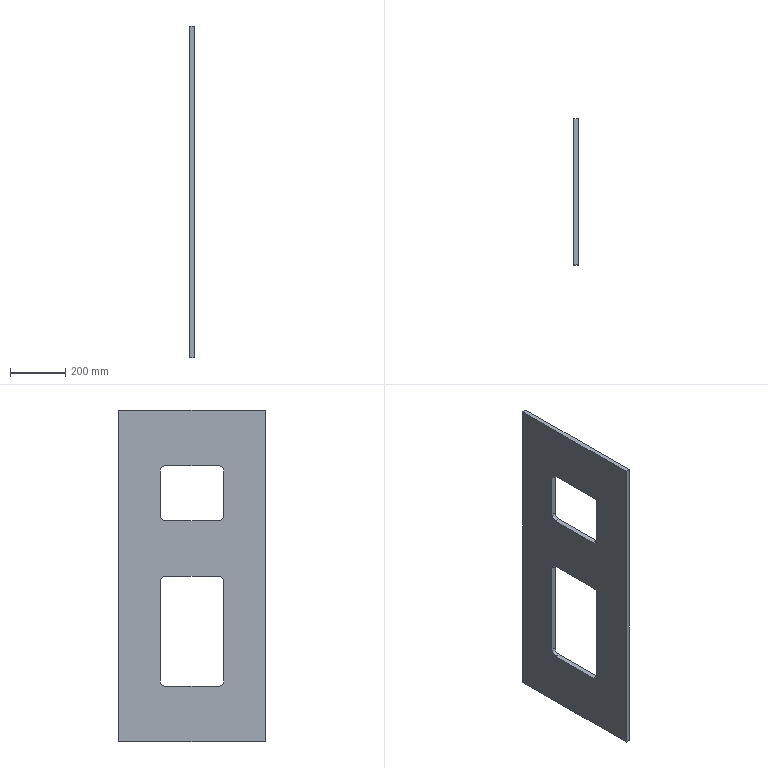Component | SolidWorks | ElectromagneticMainBeamRibPlate1-19 | 1 solid | 22 faces | box 16 x 530 x 1200 mm | volume 7978988 mm3 | plane 14 | cylinder 8 | commonest cylinder face diameters 40 x8 | material Plain Carbon Steel
STEP:
#1=COLOUR_RGB('',0.7922,0.8196,0.9333);
#2=FILL_AREA_STYLE_COLOUR('',#1);
#3=FILL_AREA_STYLE('',(#2));
#4=SURFACE_STYLE_FILL_AREA(#3);
#5=SURFACE_SIDE_STYLE('',(#4));
#6=SURFACE_STYLE_USAGE(.BOTH.,#5);
#7=PRESENTATION_STYLE_ASSIGNMENT((#6));
#8=CARTESIAN_POINT('',(-139.664,116.997,262.758));
#9=VERTEX_POINT('',#8);
#10=CARTESIAN_POINT('',(-139.664,116.997,215.514));
#11=VERTEX_POINT('',#10);
#12=CARTESIAN_POINT('',(-139.664,116.997,262.758));
#13=DIRECTION('',(-0.,0.,-1.));
#14=VECTOR('',#13,39.37);
#15=LINE('',#12,#14);
#16=EDGE_CURVE('',#9,#11,#15,.T.);
#17=ORIENTED_EDGE('',*,*,#16,.F.);
#18=CARTESIAN_POINT('',(-140.294,116.997,262.758));
#19=VERTEX_POINT('',#18);
#20=CARTESIAN_POINT('',(-140.294,116.997,262.758));
#21=DIRECTION('',(1.,0.,-0.));
#22=VECTOR('',#21,39.37);
#23=LINE('',#20,#22);
#24=EDGE_CURVE('',#19,#9,#23,.T.);
#25=ORIENTED_EDGE('',*,*,#24,.F.);
#26=CARTESIAN_POINT('',(-140.294,116.997,215.514));
#27=VERTEX_POINT('',#26);
#28=CARTESIAN_POINT('',(-140.294,116.997,262.758));
#29=DIRECTION('',(-0.,0.,-1.));
#30=VECTOR('',#29,39.37);
#31=LINE('',#28,#30);
#32=EDGE_CURVE('',#19,#27,#31,.T.);
#33=ORIENTED_EDGE('',*,*,#32,.T.);
#34=CARTESIAN_POINT('',(-140.294,116.997,215.514));
#35=DIRECTION('',(1.,0.,-0.));
#36=VECTOR('',#35,39.37);
#37=LINE('',#34,#36);
#38=EDGE_CURVE('',#27,#11,#37,.T.);
#39=ORIENTED_EDGE('',*,*,#38,.T.);
#40=EDGE_LOOP('',(#17,#25,#33,#39));
#41=FACE_OUTER_BOUND('',#40,.T.);
#42=CARTESIAN_POINT('',(-140.294,116.997,262.758));
#43=DIRECTION('',(0.,-1.,-0.));
#44=DIRECTION('',(-0.,0.,-1.));
#45=AXIS2_PLACEMENT_3D('',#42,#43,#44);
#46=PLANE('',#45);
#47=ADVANCED_FACE('',(#41),#46,.T.);
#48=CARTESIAN_POINT('',(-139.664,137.863,262.758));
#49=VERTEX_POINT('',#48);
#50=CARTESIAN_POINT('',(-139.664,116.997,262.758));
#51=DIRECTION('',(0.,-1.,0.));
#52=VECTOR('',#51,39.37);
#53=LINE('',#50,#52);
#54=EDGE_CURVE('',#49,#9,#53,.T.);
#55=ORIENTED_EDGE('',*,*,#54,.F.);
#56=CARTESIAN_POINT('',(-140.294,137.863,262.758));
#57=VERTEX_POINT('',#56);
#58=CARTESIAN_POINT('',(-140.294,137.863,262.758));
#59=DIRECTION('',(1.,0.,-0.));
#60=VECTOR('',#59,39.37);
#61=LINE('',#58,#60);
#62=EDGE_CURVE('',#57,#49,#61,.T.);
#63=ORIENTED_EDGE('',*,*,#62,.F.);
#64=CARTESIAN_POINT('',(-140.294,116.997,262.758));
#65=DIRECTION('',(0.,-1.,0.));
#66=VECTOR('',#65,39.37);
#67=LINE('',#64,#66);
#68=EDGE_CURVE('',#57,#19,#67,.T.);
#69=ORIENTED_EDGE('',*,*,#68,.T.);
#70=ORIENTED_EDGE('',*,*,#24,.T.);
#71=EDGE_LOOP('',(#55,#63,#69,#70));
#72=FACE_OUTER_BOUND('',#71,.T.);
#73=CARTESIAN_POINT('',(-140.294,116.997,262.758));
#74=DIRECTION('',(0.,0.,1.));
#75=DIRECTION('',(0.,-1.,0.));
#76=AXIS2_PLACEMENT_3D('',#73,#74,#75);
#77=PLANE('',#76);
#78=ADVANCED_FACE('',(#72),#77,.T.);
#79=CARTESIAN_POINT('',(-139.664,137.863,215.514));
#80=VERTEX_POINT('',#79);
#81=CARTESIAN_POINT('',(-139.664,137.863,262.758));
#82=DIRECTION('',(0.,-0.,1.));
#83=VECTOR('',#82,39.37);
#84=LINE('',#81,#83);
#85=EDGE_CURVE('',#80,#49,#84,.T.);
#86=ORIENTED_EDGE('',*,*,#85,.F.);
#87=CARTESIAN_POINT('',(-140.294,137.863,215.514));
#88=VERTEX_POINT('',#87);
#89=CARTESIAN_POINT('',(-140.294,137.863,215.514));
#90=DIRECTION('',(1.,0.,-0.));
#91=VECTOR('',#90,39.37);
#92=LINE('',#89,#91);
#93=EDGE_CURVE('',#88,#80,#92,.T.);
#94=ORIENTED_EDGE('',*,*,#93,.F.);
#95=CARTESIAN_POINT('',(-140.294,137.863,262.758));
#96=DIRECTION('',(0.,-0.,1.));
#97=VECTOR('',#96,39.37);
#98=LINE('',#95,#97);
#99=EDGE_CURVE('',#88,#57,#98,.T.);
#100=ORIENTED_EDGE('',*,*,#99,.T.);
#101=ORIENTED_EDGE('',*,*,#62,.T.);
#102=EDGE_LOOP('',(#86,#94,#100,#101));
#103=FACE_OUTER_BOUND('',#102,.T.);
#104=CARTESIAN_POINT('',(-140.294,137.863,262.758));
#105=DIRECTION('',(-0.,1.,0.));
#106=DIRECTION('',(0.,-0.,1.));
#107=AXIS2_PLACEMENT_3D('',#104,#105,#106);
#108=PLANE('',#107);
#109=ADVANCED_FACE('',(#103),#108,.T.);
#110=CARTESIAN_POINT('',(-139.664,116.997,215.514));
#111=DIRECTION('',(-0.,1.,0.));
#112=VECTOR('',#111,39.37);
#113=LINE('',#110,#112);
#114=EDGE_CURVE('',#11,#80,#113,.T.);
#115=ORIENTED_EDGE('',*,*,#114,.F.);
#116=ORIENTED_EDGE('',*,*,#38,.F.);
#117=CARTESIAN_POINT('',(-140.294,116.997,215.514));
#118=DIRECTION('',(-0.,1.,0.));
#119=VECTOR('',#118,39.37);
#120=LINE('',#117,#119);
#121=EDGE_CURVE('',#27,#88,#120,.T.);
#122=ORIENTED_EDGE('',*,*,#121,.T.);
#123=ORIENTED_EDGE('',*,*,#93,.T.);
#124=EDGE_LOOP('',(#115,#116,#122,#123));
#125=FACE_OUTER_BOUND('',#124,.T.);
#126=CARTESIAN_POINT('',(-140.294,116.997,215.514));
#127=DIRECTION('',(-0.,-0.,-1.));
#128=DIRECTION('',(-0.,1.,0.));
#129=AXIS2_PLACEMENT_3D('',#126,#127,#128);
#130=PLANE('',#129);
#131=ADVANCED_FACE('',(#125),#130,.T.);
#132=CARTESIAN_POINT('',(-140.294,122.903,254.096));
#133=VERTEX_POINT('',#132);
#134=CARTESIAN_POINT('',(-140.294,122.903,247.797));
#135=VERTEX_POINT('',#134);
#136=CARTESIAN_POINT('',(-140.294,122.903,254.096));
#137=DIRECTION('',(-0.,-0.,-1.));
#138=VECTOR('',#137,39.37);
#139=LINE('',#136,#138);
#140=EDGE_CURVE('',#133,#135,#139,.T.);
#141=ORIENTED_EDGE('',*,*,#140,.T.);
#142=CARTESIAN_POINT('',(-140.294,123.69,247.01));
#143=VERTEX_POINT('',#142);
#144=CARTESIAN_POINT('',(-140.294,123.69,247.797));
#145=DIRECTION('',(1.,0.,-0.));
#146=DIRECTION('',(0.,0.,-1.));
#147=AXIS2_PLACEMENT_3D('',#144,#145,#146);
#148=CIRCLE('',#147,0.7874);
#149=EDGE_CURVE('',#135,#143,#148,.T.);
#150=ORIENTED_EDGE('',*,*,#149,.T.);
#151=CARTESIAN_POINT('',(-140.294,131.171,247.01));
#152=VERTEX_POINT('',#151);
#153=CARTESIAN_POINT('',(-140.294,123.69,247.01));
#154=DIRECTION('',(-0.,1.,0.));
#155=VECTOR('',#154,39.37);
#156=LINE('',#153,#155);
#157=EDGE_CURVE('',#143,#152,#156,.T.);
#158=ORIENTED_EDGE('',*,*,#157,.T.);
#159=CARTESIAN_POINT('',(-140.294,131.958,247.797));
#160=VERTEX_POINT('',#159);
#161=CARTESIAN_POINT('',(-140.294,131.171,247.797));
#162=DIRECTION('',(1.,0.,-0.));
#163=DIRECTION('',(0.,0.,-1.));
#164=AXIS2_PLACEMENT_3D('',#161,#162,#163);
#165=CIRCLE('',#164,0.7874);
#166=EDGE_CURVE('',#152,#160,#165,.T.);
#167=ORIENTED_EDGE('',*,*,#166,.T.);
#168=CARTESIAN_POINT('',(-140.294,131.958,254.096));
#169=VERTEX_POINT('',#168);
#170=CARTESIAN_POINT('',(-140.294,131.958,254.096));
#171=DIRECTION('',(0.,0.,1.));
#172=VECTOR('',#171,39.37);
#173=LINE('',#170,#172);
#174=EDGE_CURVE('',#160,#169,#173,.T.);
#175=ORIENTED_EDGE('',*,*,#174,.T.);
#176=CARTESIAN_POINT('',(-140.294,131.171,254.884));
#177=VERTEX_POINT('',#176);
#178=CARTESIAN_POINT('',(-140.294,131.171,254.096));
#179=DIRECTION('',(1.,0.,-0.));
#180=DIRECTION('',(0.,0.,1.));
#181=AXIS2_PLACEMENT_3D('',#178,#179,#180);
#182=CIRCLE('',#181,0.7874);
#183=EDGE_CURVE('',#169,#177,#182,.T.);
#184=ORIENTED_EDGE('',*,*,#183,.T.);
#185=CARTESIAN_POINT('',(-140.294,123.69,254.884));
#186=VERTEX_POINT('',#185);
#187=CARTESIAN_POINT('',(-140.294,123.69,254.884));
#188=DIRECTION('',(0.,-1.,0.));
#189=VECTOR('',#188,39.37);
#190=LINE('',#187,#189);
#191=EDGE_CURVE('',#177,#186,#190,.T.);
#192=ORIENTED_EDGE('',*,*,#191,.T.);
#193=CARTESIAN_POINT('',(-140.294,123.69,254.096));
#194=DIRECTION('',(1.,0.,-0.));
#195=DIRECTION('',(0.,0.,-1.));
#196=AXIS2_PLACEMENT_3D('',#193,#194,#195);
#197=CIRCLE('',#196,0.7874);
#198=EDGE_CURVE('',#186,#133,#197,.T.);
#199=ORIENTED_EDGE('',*,*,#198,.T.);
#200=EDGE_LOOP('',(#141,#150,#158,#167,#175,#184,#192,#199));
#201=FACE_BOUND('',#200,.T.);
#202=CARTESIAN_POINT('',(-140.294,122.903,238.348));
#203=VERTEX_POINT('',#202);
#204=CARTESIAN_POINT('',(-140.294,122.903,224.175));
#205=VERTEX_POINT('',#204);
#206=CARTESIAN_POINT('',(-140.294,122.903,238.348));
#207=DIRECTION('',(-0.,0.,-1.));
#208=VECTOR('',#207,39.37);
#209=LINE('',#206,#208);
#210=EDGE_CURVE('',#203,#205,#209,.T.);
#211=ORIENTED_EDGE('',*,*,#210,.T.);
#212=CARTESIAN_POINT('',(-140.294,123.69,223.388));
#213=VERTEX_POINT('',#212);
#214=CARTESIAN_POINT('',(-140.294,123.69,224.175));
#215=DIRECTION('',(1.,0.,-0.));
#216=DIRECTION('',(0.,0.,-1.));
#217=AXIS2_PLACEMENT_3D('',#214,#215,#216);
#218=CIRCLE('',#217,0.7874);
#219=EDGE_CURVE('',#205,#213,#218,.T.);
#220=ORIENTED_EDGE('',*,*,#219,.T.);
#221=CARTESIAN_POINT('',(-140.294,131.171,223.388));
#222=VERTEX_POINT('',#221);
#223=CARTESIAN_POINT('',(-140.294,123.69,223.388));
#224=DIRECTION('',(-0.,1.,0.));
#225=VECTOR('',#224,39.37);
#226=LINE('',#223,#225);
#227=EDGE_CURVE('',#213,#222,#226,.T.);
#228=ORIENTED_EDGE('',*,*,#227,.T.);
#229=CARTESIAN_POINT('',(-140.294,131.958,224.175));
#230=VERTEX_POINT('',#229);
#231=CARTESIAN_POINT('',(-140.294,131.171,224.175));
#232=DIRECTION('',(1.,0.,-0.));
#233=DIRECTION('',(0.,0.,-1.));
#234=AXIS2_PLACEMENT_3D('',#231,#232,#233);
#235=CIRCLE('',#234,0.7874);
#236=EDGE_CURVE('',#222,#230,#235,.T.);
#237=ORIENTED_EDGE('',*,*,#236,.T.);
#238=CARTESIAN_POINT('',(-140.294,131.958,238.348));
#239=VERTEX_POINT('',#238);
#240=CARTESIAN_POINT('',(-140.294,131.958,238.348));
#241=DIRECTION('',(0.,0.,1.));
#242=VECTOR('',#241,39.37);
#243=LINE('',#240,#242);
#244=EDGE_CURVE('',#230,#239,#243,.T.);
#245=ORIENTED_EDGE('',*,*,#244,.T.);
#246=CARTESIAN_POINT('',(-140.294,131.171,239.136));
#247=VERTEX_POINT('',#246);
#248=CARTESIAN_POINT('',(-140.294,131.171,238.348));
#249=DIRECTION('',(1.,0.,-0.));
#250=DIRECTION('',(0.,0.,1.));
#251=AXIS2_PLACEMENT_3D('',#248,#249,#250);
#252=CIRCLE('',#251,0.7874);
#253=EDGE_CURVE('',#239,#247,#252,.T.);
#254=ORIENTED_EDGE('',*,*,#253,.T.);
#255=CARTESIAN_POINT('',(-140.294,123.69,239.136));
#256=VERTEX_POINT('',#255);
#257=CARTESIAN_POINT('',(-140.294,123.69,239.136));
#258=DIRECTION('',(0.,-1.,0.));
#259=VECTOR('',#258,39.37);
#260=LINE('',#257,#259);
#261=EDGE_CURVE('',#247,#256,#260,.T.);
#262=ORIENTED_EDGE('',*,*,#261,.T.);
#263=CARTESIAN_POINT('',(-140.294,123.69,238.348));
#264=DIRECTION('',(1.,0.,-0.));
#265=DIRECTION('',(0.,0.,-1.));
#266=AXIS2_PLACEMENT_3D('',#263,#264,#265);
#267=CIRCLE('',#266,0.7874);
#268=EDGE_CURVE('',#256,#203,#267,.T.);
#269=ORIENTED_EDGE('',*,*,#268,.T.);
#270=EDGE_LOOP('',(#211,#220,#228,#237,#245,#254,#262,#269));
#271=FACE_BOUND('',#270,.T.);
#272=ORIENTED_EDGE('',*,*,#32,.F.);
#273=ORIENTED_EDGE('',*,*,#68,.F.);
#274=ORIENTED_EDGE('',*,*,#99,.F.);
#275=ORIENTED_EDGE('',*,*,#121,.F.);
#276=EDGE_LOOP('',(#272,#273,#274,#275));
#277=FACE_OUTER_BOUND('',#276,.T.);
#278=CARTESIAN_POINT('',(-140.294,116.997,262.758));
#279=DIRECTION('',(1.,0.,-0.));
#280=DIRECTION('',(-0.,-0.,-1.));
#281=AXIS2_PLACEMENT_3D('',#278,#279,#280);
#282=PLANE('',#281);
#283=ADVANCED_FACE('',(#201,#271,#277),#282,.F.);
#284=CARTESIAN_POINT('',(-139.664,122.903,247.797));
#285=VERTEX_POINT('',#284);
#286=CARTESIAN_POINT('',(-139.664,123.69,247.01));
#287=VERTEX_POINT('',#286);
#288=CARTESIAN_POINT('',(-139.664,123.69,247.797));
#289=DIRECTION('',(1.,0.,-0.));
#290=DIRECTION('',(0.,0.,-1.));
#291=AXIS2_PLACEMENT_3D('',#288,#289,#290);
#292=CIRCLE('',#291,0.7874);
#293=EDGE_CURVE('',#285,#287,#292,.T.);
#294=ORIENTED_EDGE('',*,*,#293,.F.);
#295=CARTESIAN_POINT('',(-139.664,122.903,254.096));
#296=VERTEX_POINT('',#295);
#297=CARTESIAN_POINT('',(-139.664,122.903,254.096));
#298=DIRECTION('',(-0.,-0.,-1.));
#299=VECTOR('',#298,39.37);
#300=LINE('',#297,#299);
#301=EDGE_CURVE('',#296,#285,#300,.T.);
#302=ORIENTED_EDGE('',*,*,#301,.F.);
#303=CARTESIAN_POINT('',(-139.664,123.69,254.884));
#304=VERTEX_POINT('',#303);
#305=CARTESIAN_POINT('',(-139.664,123.69,254.096));
#306=DIRECTION('',(1.,0.,-0.));
#307=DIRECTION('',(0.,0.,-1.));
#308=AXIS2_PLACEMENT_3D('',#305,#306,#307);
#309=CIRCLE('',#308,0.7874);
#310=EDGE_CURVE('',#304,#296,#309,.T.);
#311=ORIENTED_EDGE('',*,*,#310,.F.);
#312=CARTESIAN_POINT('',(-139.664,131.171,254.884));
#313=VERTEX_POINT('',#312);
#314=CARTESIAN_POINT('',(-139.664,123.69,254.884));
#315=DIRECTION('',(0.,-1.,0.));
#316=VECTOR('',#315,39.37);
#317=LINE('',#314,#316);
#318=EDGE_CURVE('',#313,#304,#317,.T.);
#319=ORIENTED_EDGE('',*,*,#318,.F.);
#320=CARTESIAN_POINT('',(-139.664,131.958,254.096));
#321=VERTEX_POINT('',#320);
#322=CARTESIAN_POINT('',(-139.664,131.171,254.096));
#323=DIRECTION('',(1.,0.,-0.));
#324=DIRECTION('',(0.,0.,1.));
#325=AXIS2_PLACEMENT_3D('',#322,#323,#324);
#326=CIRCLE('',#325,0.7874);
#327=EDGE_CURVE('',#321,#313,#326,.T.);
#328=ORIENTED_EDGE('',*,*,#327,.F.);
#329=CARTESIAN_POINT('',(-139.664,131.958,247.797));
#330=VERTEX_POINT('',#329);
#331=CARTESIAN_POINT('',(-139.664,131.958,254.096));
#332=DIRECTION('',(0.,0.,1.));
#333=VECTOR('',#332,39.37);
#334=LINE('',#331,#333);
#335=EDGE_CURVE('',#330,#321,#334,.T.);
#336=ORIENTED_EDGE('',*,*,#335,.F.);
#337=CARTESIAN_POINT('',(-139.664,131.171,247.01));
#338=VERTEX_POINT('',#337);
#339=CARTESIAN_POINT('',(-139.664,131.171,247.797));
#340=DIRECTION('',(1.,0.,-0.));
#341=DIRECTION('',(0.,0.,-1.));
#342=AXIS2_PLACEMENT_3D('',#339,#340,#341);
#343=CIRCLE('',#342,0.7874);
#344=EDGE_CURVE('',#338,#330,#343,.T.);
#345=ORIENTED_EDGE('',*,*,#344,.F.);
#346=CARTESIAN_POINT('',(-139.664,123.69,247.01));
#347=DIRECTION('',(-0.,1.,0.));
#348=VECTOR('',#347,39.37);
#349=LINE('',#346,#348);
#350=EDGE_CURVE('',#287,#338,#349,.T.);
#351=ORIENTED_EDGE('',*,*,#350,.F.);
#352=EDGE_LOOP('',(#294,#302,#311,#319,#328,#336,#345,#351));
#353=FACE_BOUND('',#352,.T.);
#354=CARTESIAN_POINT('',(-139.664,122.903,224.175));
#355=VERTEX_POINT('',#354);
#356=CARTESIAN_POINT('',(-139.664,123.69,223.388));
#357=VERTEX_POINT('',#356);
#358=CARTESIAN_POINT('',(-139.664,123.69,224.175));
#359=DIRECTION('',(1.,0.,-0.));
#360=DIRECTION('',(0.,0.,-1.));
#361=AXIS2_PLACEMENT_3D('',#358,#359,#360);
#362=CIRCLE('',#361,0.7874);
#363=EDGE_CURVE('',#355,#357,#362,.T.);
#364=ORIENTED_EDGE('',*,*,#363,.F.);
#365=CARTESIAN_POINT('',(-139.664,122.903,238.348));
#366=VERTEX_POINT('',#365);
#367=CARTESIAN_POINT('',(-139.664,122.903,238.348));
#368=DIRECTION('',(-0.,0.,-1.));
#369=VECTOR('',#368,39.37);
#370=LINE('',#367,#369);
#371=EDGE_CURVE('',#366,#355,#370,.T.);
#372=ORIENTED_EDGE('',*,*,#371,.F.);
#373=CARTESIAN_POINT('',(-139.664,123.69,239.136));
#374=VERTEX_POINT('',#373);
#375=CARTESIAN_POINT('',(-139.664,123.69,238.348));
#376=DIRECTION('',(1.,0.,-0.));
#377=DIRECTION('',(0.,0.,-1.));
#378=AXIS2_PLACEMENT_3D('',#375,#376,#377);
#379=CIRCLE('',#378,0.7874);
#380=EDGE_CURVE('',#374,#366,#379,.T.);
#381=ORIENTED_EDGE('',*,*,#380,.F.);
#382=CARTESIAN_POINT('',(-139.664,131.171,239.136));
#383=VERTEX_POINT('',#382);
#384=CARTESIAN_POINT('',(-139.664,123.69,239.136));
#385=DIRECTION('',(0.,-1.,0.));
#386=VECTOR('',#385,39.37);
#387=LINE('',#384,#386);
#388=EDGE_CURVE('',#383,#374,#387,.T.);
#389=ORIENTED_EDGE('',*,*,#388,.F.);
#390=CARTESIAN_POINT('',(-139.664,131.958,238.348));
#391=VERTEX_POINT('',#390);
#392=CARTESIAN_POINT('',(-139.664,131.171,238.348));
#393=DIRECTION('',(1.,0.,-0.));
#394=DIRECTION('',(0.,0.,1.));
#395=AXIS2_PLACEMENT_3D('',#392,#393,#394);
#396=CIRCLE('',#395,0.7874);
#397=EDGE_CURVE('',#391,#383,#396,.T.);
#398=ORIENTED_EDGE('',*,*,#397,.F.);
#399=CARTESIAN_POINT('',(-139.664,131.958,224.175));
#400=VERTEX_POINT('',#399);
#401=CARTESIAN_POINT('',(-139.664,131.958,238.348));
#402=DIRECTION('',(0.,0.,1.));
#403=VECTOR('',#402,39.37);
#404=LINE('',#401,#403);
#405=EDGE_CURVE('',#400,#391,#404,.T.);
#406=ORIENTED_EDGE('',*,*,#405,.F.);
#407=CARTESIAN_POINT('',(-139.664,131.171,223.388));
#408=VERTEX_POINT('',#407);
#409=CARTESIAN_POINT('',(-139.664,131.171,224.175));
#410=DIRECTION('',(1.,0.,-0.));
#411=DIRECTION('',(0.,0.,-1.));
#412=AXIS2_PLACEMENT_3D('',#409,#410,#411);
#413=CIRCLE('',#412,0.7874);
#414=EDGE_CURVE('',#408,#400,#413,.T.);
#415=ORIENTED_EDGE('',*,*,#414,.F.);
#416=CARTESIAN_POINT('',(-139.664,123.69,223.388));
#417=DIRECTION('',(-0.,1.,0.));
#418=VECTOR('',#417,39.37);
#419=LINE('',#416,#418);
#420=EDGE_CURVE('',#357,#408,#419,.T.);
#421=ORIENTED_EDGE('',*,*,#420,.F.);
#422=EDGE_LOOP('',(#364,#372,#381,#389,#398,#406,#415,#421));
#423=FACE_BOUND('',#422,.T.);
#424=ORIENTED_EDGE('',*,*,#16,.T.);
#425=ORIENTED_EDGE('',*,*,#114,.T.);
#426=ORIENTED_EDGE('',*,*,#85,.T.);
#427=ORIENTED_EDGE('',*,*,#54,.T.);
#428=EDGE_LOOP('',(#424,#425,#426,#427));
#429=FACE_OUTER_BOUND('',#428,.T.);
#430=CARTESIAN_POINT('',(-139.664,116.997,262.758));
#431=DIRECTION('',(1.,0.,-0.));
#432=DIRECTION('',(-0.,-0.,-1.));
#433=AXIS2_PLACEMENT_3D('',#430,#431,#432);
#434=PLANE('',#433);
#435=ADVANCED_FACE('',(#353,#423,#429),#434,.T.);
#436=ORIENTED_EDGE('',*,*,#363,.T.);
#437=CARTESIAN_POINT('',(-140.294,123.69,223.388));
#438=DIRECTION('',(1.,0.,-0.));
#439=VECTOR('',#438,39.37);
#440=LINE('',#437,#439);
#441=EDGE_CURVE('',#213,#357,#440,.T.);
#442=ORIENTED_EDGE('',*,*,#441,.F.);
#443=ORIENTED_EDGE('',*,*,#219,.F.);
#444=CARTESIAN_POINT('',(-140.294,122.903,224.175));
#445=DIRECTION('',(1.,0.,-0.));
#446=VECTOR('',#445,39.37);
#447=LINE('',#444,#446);
#448=EDGE_CURVE('',#205,#355,#447,.T.);
#449=ORIENTED_EDGE('',*,*,#448,.T.);
#450=EDGE_LOOP('',(#436,#442,#443,#449));
#451=FACE_OUTER_BOUND('',#450,.T.);
#452=CARTESIAN_POINT('',(-140.294,123.69,224.175));
#453=DIRECTION('',(1.,0.,-0.));
#454=DIRECTION('',(0.,0.,-1.));
#455=AXIS2_PLACEMENT_3D('',#452,#453,#454);
#456=CYLINDRICAL_SURFACE('',#455,0.7874);
#457=ADVANCED_FACE('',(#451),#456,.F.);
#458=ORIENTED_EDGE('',*,*,#371,.T.);
#459=ORIENTED_EDGE('',*,*,#448,.F.);
#460=ORIENTED_EDGE('',*,*,#210,.F.);
#461=CARTESIAN_POINT('',(-140.294,122.903,238.348));
#462=DIRECTION('',(1.,0.,-0.));
#463=VECTOR('',#462,39.37);
#464=LINE('',#461,#463);
#465=EDGE_CURVE('',#203,#366,#464,.T.);
#466=ORIENTED_EDGE('',*,*,#465,.T.);
#467=EDGE_LOOP('',(#458,#459,#460,#466));
#468=FACE_OUTER_BOUND('',#467,.T.);
#469=CARTESIAN_POINT('',(-140.294,122.903,238.348));
#470=DIRECTION('',(0.,-1.,-0.));
#471=DIRECTION('',(-0.,0.,-1.));
#472=AXIS2_PLACEMENT_3D('',#469,#470,#471);
#473=PLANE('',#472);
#474=ADVANCED_FACE('',(#468),#473,.F.);
#475=ORIENTED_EDGE('',*,*,#380,.T.);
#476=ORIENTED_EDGE('',*,*,#465,.F.);
#477=ORIENTED_EDGE('',*,*,#268,.F.);
#478=CARTESIAN_POINT('',(-140.294,123.69,239.136));
#479=DIRECTION('',(1.,0.,-0.));
#480=VECTOR('',#479,39.37);
#481=LINE('',#478,#480);
#482=EDGE_CURVE('',#256,#374,#481,.T.);
#483=ORIENTED_EDGE('',*,*,#482,.T.);
#484=EDGE_LOOP('',(#475,#476,#477,#483));
#485=FACE_OUTER_BOUND('',#484,.T.);
#486=CARTESIAN_POINT('',(-140.294,123.69,238.348));
#487=DIRECTION('',(1.,0.,-0.));
#488=DIRECTION('',(0.,0.,-1.));
#489=AXIS2_PLACEMENT_3D('',#486,#487,#488);
#490=CYLINDRICAL_SURFACE('',#489,0.7874);
#491=ADVANCED_FACE('',(#485),#490,.F.);
#492=ORIENTED_EDGE('',*,*,#388,.T.);
#493=ORIENTED_EDGE('',*,*,#482,.F.);
#494=ORIENTED_EDGE('',*,*,#261,.F.);
#495=CARTESIAN_POINT('',(-140.294,131.171,239.136));
#496=DIRECTION('',(1.,0.,-0.));
#497=VECTOR('',#496,39.37);
#498=LINE('',#495,#497);
#499=EDGE_CURVE('',#247,#383,#498,.T.);
#500=ORIENTED_EDGE('',*,*,#499,.T.);
#501=EDGE_LOOP('',(#492,#493,#494,#500));
#502=FACE_OUTER_BOUND('',#501,.T.);
#503=CARTESIAN_POINT('',(-140.294,123.69,239.136));
#504=DIRECTION('',(0.,0.,1.));
#505=DIRECTION('',(0.,-1.,0.));
#506=AXIS2_PLACEMENT_3D('',#503,#504,#505);
#507=PLANE('',#506);
#508=ADVANCED_FACE('',(#502),#507,.F.);
#509=ORIENTED_EDGE('',*,*,#397,.T.);
#510=ORIENTED_EDGE('',*,*,#499,.F.);
#511=ORIENTED_EDGE('',*,*,#253,.F.);
#512=CARTESIAN_POINT('',(-140.294,131.958,238.348));
#513=DIRECTION('',(1.,0.,-0.));
#514=VECTOR('',#513,39.37);
#515=LINE('',#512,#514);
#516=EDGE_CURVE('',#239,#391,#515,.T.);
#517=ORIENTED_EDGE('',*,*,#516,.T.);
#518=EDGE_LOOP('',(#509,#510,#511,#517));
#519=FACE_OUTER_BOUND('',#518,.T.);
#520=CARTESIAN_POINT('',(-140.294,131.171,238.348));
#521=DIRECTION('',(1.,0.,-0.));
#522=DIRECTION('',(0.,0.,-1.));
#523=AXIS2_PLACEMENT_3D('',#520,#521,#522);
#524=CYLINDRICAL_SURFACE('',#523,0.7874);
#525=ADVANCED_FACE('',(#519),#524,.F.);
#526=ORIENTED_EDGE('',*,*,#405,.T.);
#527=ORIENTED_EDGE('',*,*,#516,.F.);
#528=ORIENTED_EDGE('',*,*,#244,.F.);
#529=CARTESIAN_POINT('',(-140.294,131.958,224.175));
#530=DIRECTION('',(1.,0.,-0.));
#531=VECTOR('',#530,39.37);
#532=LINE('',#529,#531);
#533=EDGE_CURVE('',#230,#400,#532,.T.);
#534=ORIENTED_EDGE('',*,*,#533,.T.);
#535=EDGE_LOOP('',(#526,#527,#528,#534));
#536=FACE_OUTER_BOUND('',#535,.T.);
#537=CARTESIAN_POINT('',(-140.294,131.958,238.348));
#538=DIRECTION('',(-0.,1.,-0.));
#539=DIRECTION('',(0.,0.,1.));
#540=AXIS2_PLACEMENT_3D('',#537,#538,#539);
#541=PLANE('',#540);
#542=ADVANCED_FACE('',(#536),#541,.F.);
#543=ORIENTED_EDGE('',*,*,#414,.T.);
#544=ORIENTED_EDGE('',*,*,#533,.F.);
#545=ORIENTED_EDGE('',*,*,#236,.F.);
#546=CARTESIAN_POINT('',(-140.294,131.171,223.388));
#547=DIRECTION('',(1.,0.,-0.));
#548=VECTOR('',#547,39.37);
#549=LINE('',#546,#548);
#550=EDGE_CURVE('',#222,#408,#549,.T.);
#551=ORIENTED_EDGE('',*,*,#550,.T.);
#552=EDGE_LOOP('',(#543,#544,#545,#551));
#553=FACE_OUTER_BOUND('',#552,.T.);
#554=CARTESIAN_POINT('',(-140.294,131.171,224.175));
#555=DIRECTION('',(1.,0.,-0.));
#556=DIRECTION('',(0.,0.,-1.));
#557=AXIS2_PLACEMENT_3D('',#554,#555,#556);
#558=CYLINDRICAL_SURFACE('',#557,0.7874);
#559=ADVANCED_FACE('',(#553),#558,.F.);
#560=ORIENTED_EDGE('',*,*,#420,.T.);
#561=ORIENTED_EDGE('',*,*,#550,.F.);
#562=ORIENTED_EDGE('',*,*,#227,.F.);
#563=ORIENTED_EDGE('',*,*,#441,.T.);
#564=EDGE_LOOP('',(#560,#561,#562,#563));
#565=FACE_OUTER_BOUND('',#564,.T.);
#566=CARTESIAN_POINT('',(-140.294,123.69,223.388));
#567=DIRECTION('',(-0.,-0.,-1.));
#568=DIRECTION('',(-0.,1.,0.));
#569=AXIS2_PLACEMENT_3D('',#566,#567,#568);
#570=PLANE('',#569);
#571=ADVANCED_FACE('',(#565),#570,.F.);
#572=ORIENTED_EDGE('',*,*,#293,.T.);
#573=CARTESIAN_POINT('',(-140.294,123.69,247.01));
#574=DIRECTION('',(1.,0.,-0.));
#575=VECTOR('',#574,39.37);
#576=LINE('',#573,#575);
#577=EDGE_CURVE('',#143,#287,#576,.T.);
#578=ORIENTED_EDGE('',*,*,#577,.F.);
#579=ORIENTED_EDGE('',*,*,#149,.F.);
#580=CARTESIAN_POINT('',(-140.294,122.903,247.797));
#581=DIRECTION('',(1.,0.,-0.));
#582=VECTOR('',#581,39.37);
#583=LINE('',#580,#582);
#584=EDGE_CURVE('',#135,#285,#583,.T.);
#585=ORIENTED_EDGE('',*,*,#584,.T.);
#586=EDGE_LOOP('',(#572,#578,#579,#585));
#587=FACE_OUTER_BOUND('',#586,.T.);
#588=CARTESIAN_POINT('',(-140.294,123.69,247.797));
#589=DIRECTION('',(1.,0.,-0.));
#590=DIRECTION('',(0.,0.,-1.));
#591=AXIS2_PLACEMENT_3D('',#588,#589,#590);
#592=CYLINDRICAL_SURFACE('',#591,0.7874);
#593=ADVANCED_FACE('',(#587),#592,.F.);
#594=ORIENTED_EDGE('',*,*,#301,.T.);
#595=ORIENTED_EDGE('',*,*,#584,.F.);
#596=ORIENTED_EDGE('',*,*,#140,.F.);
#597=CARTESIAN_POINT('',(-140.294,122.903,254.096));
#598=DIRECTION('',(1.,0.,-0.));
#599=VECTOR('',#598,39.37);
#600=LINE('',#597,#599);
#601=EDGE_CURVE('',#133,#296,#600,.T.);
#602=ORIENTED_EDGE('',*,*,#601,.T.);
#603=EDGE_LOOP('',(#594,#595,#596,#602));
#604=FACE_OUTER_BOUND('',#603,.T.);
#605=CARTESIAN_POINT('',(-140.294,122.903,254.096));
#606=DIRECTION('',(0.,-1.,0.));
#607=DIRECTION('',(-0.,-0.,-1.));
#608=AXIS2_PLACEMENT_3D('',#605,#606,#607);
#609=PLANE('',#608);
#610=ADVANCED_FACE('',(#604),#609,.F.);
#611=ORIENTED_EDGE('',*,*,#310,.T.);
#612=ORIENTED_EDGE('',*,*,#601,.F.);
#613=ORIENTED_EDGE('',*,*,#198,.F.);
#614=CARTESIAN_POINT('',(-140.294,123.69,254.884));
#615=DIRECTION('',(1.,0.,-0.));
#616=VECTOR('',#615,39.37);
#617=LINE('',#614,#616);
#618=EDGE_CURVE('',#186,#304,#617,.T.);
#619=ORIENTED_EDGE('',*,*,#618,.T.);
#620=EDGE_LOOP('',(#611,#612,#613,#619));
#621=FACE_OUTER_BOUND('',#620,.T.);
#622=CARTESIAN_POINT('',(-140.294,123.69,254.096));
#623=DIRECTION('',(1.,0.,-0.));
#624=DIRECTION('',(0.,0.,-1.));
#625=AXIS2_PLACEMENT_3D('',#622,#623,#624);
#626=CYLINDRICAL_SURFACE('',#625,0.7874);
#627=ADVANCED_FACE('',(#621),#626,.F.);
#628=ORIENTED_EDGE('',*,*,#318,.T.);
#629=ORIENTED_EDGE('',*,*,#618,.F.);
#630=ORIENTED_EDGE('',*,*,#191,.F.);
#631=CARTESIAN_POINT('',(-140.294,131.171,254.884));
#632=DIRECTION('',(1.,0.,-0.));
#633=VECTOR('',#632,39.37);
#634=LINE('',#631,#633);
#635=EDGE_CURVE('',#177,#313,#634,.T.);
#636=ORIENTED_EDGE('',*,*,#635,.T.);
#637=EDGE_LOOP('',(#628,#629,#630,#636));
#638=FACE_OUTER_BOUND('',#637,.T.);
#639=CARTESIAN_POINT('',(-140.294,123.69,254.884));
#640=DIRECTION('',(0.,0.,1.));
#641=DIRECTION('',(0.,-1.,0.));
#642=AXIS2_PLACEMENT_3D('',#639,#640,#641);
#643=PLANE('',#642);
#644=ADVANCED_FACE('',(#638),#643,.F.);
#645=ORIENTED_EDGE('',*,*,#327,.T.);
#646=ORIENTED_EDGE('',*,*,#635,.F.);
#647=ORIENTED_EDGE('',*,*,#183,.F.);
#648=CARTESIAN_POINT('',(-140.294,131.958,254.096));
#649=DIRECTION('',(1.,0.,-0.));
#650=VECTOR('',#649,39.37);
#651=LINE('',#648,#650);
#652=EDGE_CURVE('',#169,#321,#651,.T.);
#653=ORIENTED_EDGE('',*,*,#652,.T.);
#654=EDGE_LOOP('',(#645,#646,#647,#653));
#655=FACE_OUTER_BOUND('',#654,.T.);
#656=CARTESIAN_POINT('',(-140.294,131.171,254.096));
#657=DIRECTION('',(1.,0.,-0.));
#658=DIRECTION('',(0.,0.,-1.));
#659=AXIS2_PLACEMENT_3D('',#656,#657,#658);
#660=CYLINDRICAL_SURFACE('',#659,0.7874);
#661=ADVANCED_FACE('',(#655),#660,.F.);
#662=ORIENTED_EDGE('',*,*,#335,.T.);
#663=ORIENTED_EDGE('',*,*,#652,.F.);
#664=ORIENTED_EDGE('',*,*,#174,.F.);
#665=CARTESIAN_POINT('',(-140.294,131.958,247.797));
#666=DIRECTION('',(1.,0.,-0.));
#667=VECTOR('',#666,39.37);
#668=LINE('',#665,#667);
#669=EDGE_CURVE('',#160,#330,#668,.T.);
#670=ORIENTED_EDGE('',*,*,#669,.T.);
#671=EDGE_LOOP('',(#662,#663,#664,#670));
#672=FACE_OUTER_BOUND('',#671,.T.);
#673=CARTESIAN_POINT('',(-140.294,131.958,254.096));
#674=DIRECTION('',(-0.,1.,-0.));
#675=DIRECTION('',(0.,0.,1.));
#676=AXIS2_PLACEMENT_3D('',#673,#674,#675);
#677=PLANE('',#676);
#678=ADVANCED_FACE('',(#672),#677,.F.);
#679=ORIENTED_EDGE('',*,*,#344,.T.);
#680=ORIENTED_EDGE('',*,*,#669,.F.);
#681=ORIENTED_EDGE('',*,*,#166,.F.);
#682=CARTESIAN_POINT('',(-140.294,131.171,247.01));
#683=DIRECTION('',(1.,0.,-0.));
#684=VECTOR('',#683,39.37);
#685=LINE('',#682,#684);
#686=EDGE_CURVE('',#152,#338,#685,.T.);
#687=ORIENTED_EDGE('',*,*,#686,.T.);
#688=EDGE_LOOP('',(#679,#680,#681,#687));
#689=FACE_OUTER_BOUND('',#688,.T.);
#690=CARTESIAN_POINT('',(-140.294,131.171,247.797));
#691=DIRECTION('',(1.,0.,-0.));
#692=DIRECTION('',(0.,0.,-1.));
#693=AXIS2_PLACEMENT_3D('',#690,#691,#692);
#694=CYLINDRICAL_SURFACE('',#693,0.7874);
#695=ADVANCED_FACE('',(#689),#694,.F.);
#696=ORIENTED_EDGE('',*,*,#350,.T.);
#697=ORIENTED_EDGE('',*,*,#686,.F.);
#698=ORIENTED_EDGE('',*,*,#157,.F.);
#699=ORIENTED_EDGE('',*,*,#577,.T.);
#700=EDGE_LOOP('',(#696,#697,#698,#699));
#701=FACE_OUTER_BOUND('',#700,.T.);
#702=CARTESIAN_POINT('',(-140.294,123.69,247.01));
#703=DIRECTION('',(-0.,-0.,-1.));
#704=DIRECTION('',(-0.,1.,0.));
#705=AXIS2_PLACEMENT_3D('',#702,#703,#704);
#706=PLANE('',#705);
#707=ADVANCED_FACE('',(#701),#706,.F.);
#708=CLOSED_SHELL('',(#47,#78,#109,#131,#283,#435,#457,#474,#491,#508,#525,#542,#559,#571,#593,#610,#627,#644,#661,#678,#695,#707));
#709=MANIFOLD_SOLID_BREP('',#708);
#710=STYLED_ITEM('',(#7),#709);
#711=PRESENTATION_LAYER_ASSIGNMENT('','',(#710));
#712=(LENGTH_UNIT()NAMED_UNIT(*)SI_UNIT($,.METRE.));
#713=LENGTH_MEASURE_WITH_UNIT(LENGTH_MEASURE(0.0254),#712);
#714=DIMENSIONAL_EXPONENTS(1.,0.,0.,0.,0.,0.,0.);
#715=(CONVERSION_BASED_UNIT('',#713)LENGTH_UNIT()NAMED_UNIT(#714));
#716=UNCERTAINTY_MEASURE_WITH_UNIT(LENGTH_MEASURE(0.00001),#715,'','');
#717=(NAMED_UNIT(*)PLANE_ANGLE_UNIT()SI_UNIT($,.RADIAN.));
#718=(NAMED_UNIT(*)SI_UNIT($,.STERADIAN.)SOLID_ANGLE_UNIT());
#719=(GEOMETRIC_REPRESENTATION_CONTEXT(3)GLOBAL_UNCERTAINTY_ASSIGNED_CONTEXT((#716))GLOBAL_UNIT_ASSIGNED_CONTEXT((#715,#717,#718))REPRESENTATION_CONTEXT('',''));
#720=MECHANICAL_DESIGN_GEOMETRIC_PRESENTATION_REPRESENTATION('',(#710),#719);
#721=CARTESIAN_POINT('',(0.,0.,0.));
#722=DIRECTION('',(0.,0.,1.));
#723=DIRECTION('',(1.,0.,0.));
#724=AXIS2_PLACEMENT_3D('',#721,#722,#723);
#725=(LENGTH_UNIT()NAMED_UNIT(*)SI_UNIT($,.METRE.));
#726=LENGTH_MEASURE_WITH_UNIT(LENGTH_MEASURE(0.0254),#725);
#727=DIMENSIONAL_EXPONENTS(1.,0.,0.,0.,0.,0.,0.);
#728=(CONVERSION_BASED_UNIT('',#726)LENGTH_UNIT()NAMED_UNIT(#727));
#729=UNCERTAINTY_MEASURE_WITH_UNIT(LENGTH_MEASURE(0.00001),#728,'','');
#730=(NAMED_UNIT(*)PLANE_ANGLE_UNIT()SI_UNIT($,.RADIAN.));
#731=(NAMED_UNIT(*)SI_UNIT($,.STERADIAN.)SOLID_ANGLE_UNIT());
#732=(GEOMETRIC_REPRESENTATION_CONTEXT(3)GLOBAL_UNCERTAINTY_ASSIGNED_CONTEXT((#729))GLOBAL_UNIT_ASSIGNED_CONTEXT((#728,#730,#731))REPRESENTATION_CONTEXT('',''));
#733=ADVANCED_BREP_SHAPE_REPRESENTATION('',(#709,#724),#732);